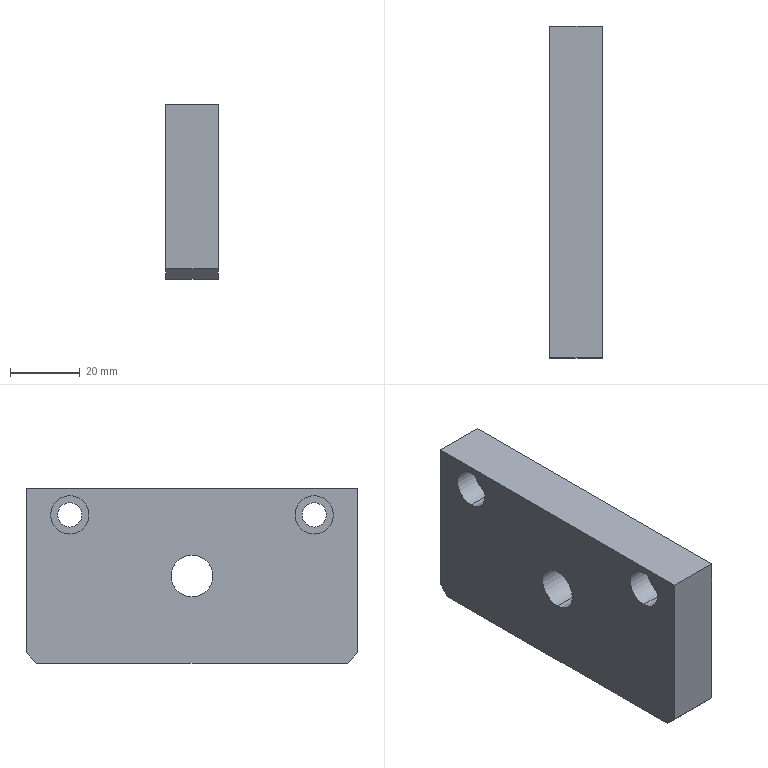Component | SolidWorks | -TighteningHandwheelBasePlate-2 | 1 solid | 20 faces | box 15 x 95 x 50 mm | volume 67472 mm3 | cylinder 10 | plane 10 | commonest cylinder face diameters 11 x4 7 x4 12 x2
build123d program:
from build123d import *

# Parameters (mm, degrees)
SKETCH1_W                                           = 50
SKETCH1_H                                           = 95
BOSS_EXTRUDE1_DEPTH                                 = 15
SKETCH2_R                                           = 6
CUT_EXTRUDE1_DEPTH                                  = 56.734
CYLINDRICAL_COUNTERSUNK_HOLE_FOR_M6_HEX_D           = 7
CYLINDRICAL_COUNTERSUNK_HOLE_FOR_M6_HEX_CBORE_D     = 11
CYLINDRICAL_COUNTERSUNK_HOLE_FOR_M6_HEX_CBORE_DEPTH = 7
CHAMFER1_SIZE                                       = 3


with BuildPart() as part:
    # Sketch1 → Boss-Extrude1 (new body)
    with BuildSketch(Plane.XY):
        Rectangle(SKETCH1_W, SKETCH1_H)
    extrude(amount=BOSS_EXTRUDE1_DEPTH)

    # Sketch2 → Cut-Extrude1 (cut, through all)
    with BuildSketch(Plane.XY.offset(15)):
        Circle(SKETCH2_R)
    extrude(amount=-CUT_EXTRUDE1_DEPTH, mode=Mode.SUBTRACT)

    # Cylindrical Countersunk Hole for M6 Hex (through all)
    with Locations(Plane.XY.offset(15)):
        with Locations((-17.5, 35), (-17.5, -35)):
            CounterBoreHole(CYLINDRICAL_COUNTERSUNK_HOLE_FOR_M6_HEX_D / 2, CYLINDRICAL_COUNTERSUNK_HOLE_FOR_M6_HEX_CBORE_D / 2, CYLINDRICAL_COUNTERSUNK_HOLE_FOR_M6_HEX_CBORE_DEPTH)

    # Chamfer1
    chamfer1_edges = [part.edges().sort_by_distance(p)[0] for p in [
        (25, -47.5, 7.5),
        (25, 47.5, 7.5),
    ]]
    chamfer(chamfer1_edges, length=CHAMFER1_SIZE)


solid = part.part

# Placed as in the assembly
solid = solid.moved(Location((-260, 1239.5, -20), (180, -90, 0)))
STEP:
#1=COLOUR_RGB('',0.7922,0.8196,0.9333);
#2=FILL_AREA_STYLE_COLOUR('',#1);
#3=FILL_AREA_STYLE('',(#2));
#4=SURFACE_STYLE_FILL_AREA(#3);
#5=SURFACE_SIDE_STYLE('',(#4));
#6=SURFACE_STYLE_USAGE(.BOTH.,#5);
#7=PRESENTATION_STYLE_ASSIGNMENT((#6));
#8=CARTESIAN_POINT('',(-10.551,47.421,0.1181));
#9=VERTEX_POINT('',#8);
#10=CARTESIAN_POINT('',(-10.551,47.421,-0.315));
#11=VERTEX_POINT('',#10);
#12=CARTESIAN_POINT('',(-10.551,47.421,-0.09843));
#13=DIRECTION('',(-1.,-0.,0.));
#14=DIRECTION('',(0.,0.,-1.));
#15=AXIS2_PLACEMENT_3D('',#12,#13,#14);
#16=CIRCLE('',#15,0.2165);
#17=EDGE_CURVE('',#9,#11,#16,.T.);
#18=ORIENTED_EDGE('',*,*,#17,.F.);
#19=CARTESIAN_POINT('',(-10.827,47.421,0.1181));
#20=VERTEX_POINT('',#19);
#21=CARTESIAN_POINT('',(-10.827,47.421,0.1181));
#22=DIRECTION('',(-1.,-0.,0.));
#23=VECTOR('',#22,39.37);
#24=LINE('',#21,#23);
#25=EDGE_CURVE('',#9,#20,#24,.T.);
#26=ORIENTED_EDGE('',*,*,#25,.T.);
#27=CARTESIAN_POINT('',(-10.827,47.421,-0.315));
#28=VERTEX_POINT('',#27);
#29=CARTESIAN_POINT('',(-10.827,47.421,-0.09843));
#30=DIRECTION('',(-1.,-0.,0.));
#31=DIRECTION('',(0.,0.,-1.));
#32=AXIS2_PLACEMENT_3D('',#29,#30,#31);
#33=CIRCLE('',#32,0.2165);
#34=EDGE_CURVE('',#20,#28,#33,.T.);
#35=ORIENTED_EDGE('',*,*,#34,.T.);
#36=CARTESIAN_POINT('',(-10.827,47.421,-0.315));
#37=DIRECTION('',(-1.,-0.,0.));
#38=VECTOR('',#37,39.37);
#39=LINE('',#36,#38);
#40=EDGE_CURVE('',#11,#28,#39,.T.);
#41=ORIENTED_EDGE('',*,*,#40,.F.);
#42=EDGE_LOOP('',(#18,#26,#35,#41));
#43=FACE_OUTER_BOUND('',#42,.T.);
#44=CARTESIAN_POINT('',(-10.827,47.421,-0.09843));
#45=DIRECTION('',(-1.,-0.,0.));
#46=DIRECTION('',(0.,0.,-1.));
#47=AXIS2_PLACEMENT_3D('',#44,#45,#46);
#48=CYLINDRICAL_SURFACE('',#47,0.2165);
#49=ADVANCED_FACE('',(#43),#48,.F.);
#50=CARTESIAN_POINT('',(-10.236,47.421,0.03937));
#51=VERTEX_POINT('',#50);
#52=CARTESIAN_POINT('',(-10.236,47.421,-0.2362));
#53=VERTEX_POINT('',#52);
#54=CARTESIAN_POINT('',(-10.236,47.421,-0.09843));
#55=DIRECTION('',(-1.,-0.,0.));
#56=DIRECTION('',(0.,0.,-1.));
#57=AXIS2_PLACEMENT_3D('',#54,#55,#56);
#58=CIRCLE('',#57,0.1378);
#59=EDGE_CURVE('',#51,#53,#58,.T.);
#60=ORIENTED_EDGE('',*,*,#59,.F.);
#61=CARTESIAN_POINT('',(-10.551,47.421,0.03937));
#62=VERTEX_POINT('',#61);
#63=CARTESIAN_POINT('',(-10.827,47.421,0.03937));
#64=DIRECTION('',(-1.,-0.,0.));
#65=VECTOR('',#64,39.37);
#66=LINE('',#63,#65);
#67=EDGE_CURVE('',#51,#62,#66,.T.);
#68=ORIENTED_EDGE('',*,*,#67,.T.);
#69=CARTESIAN_POINT('',(-10.551,47.421,-0.2362));
#70=VERTEX_POINT('',#69);
#71=CARTESIAN_POINT('',(-10.551,47.421,-0.09843));
#72=DIRECTION('',(-1.,-0.,0.));
#73=DIRECTION('',(0.,0.,-1.));
#74=AXIS2_PLACEMENT_3D('',#71,#72,#73);
#75=CIRCLE('',#74,0.1378);
#76=EDGE_CURVE('',#62,#70,#75,.T.);
#77=ORIENTED_EDGE('',*,*,#76,.T.);
#78=CARTESIAN_POINT('',(-10.827,47.421,-0.2362));
#79=DIRECTION('',(-1.,-0.,0.));
#80=VECTOR('',#79,39.37);
#81=LINE('',#78,#80);
#82=EDGE_CURVE('',#53,#70,#81,.T.);
#83=ORIENTED_EDGE('',*,*,#82,.F.);
#84=EDGE_LOOP('',(#60,#68,#77,#83));
#85=FACE_OUTER_BOUND('',#84,.T.);
#86=CARTESIAN_POINT('',(-10.827,47.421,-0.09843));
#87=DIRECTION('',(-1.,-0.,0.));
#88=DIRECTION('',(0.,0.,-1.));
#89=AXIS2_PLACEMENT_3D('',#86,#87,#88);
#90=CYLINDRICAL_SURFACE('',#89,0.1378);
#91=ADVANCED_FACE('',(#85),#90,.F.);
#92=CARTESIAN_POINT('',(-10.551,50.177,0.1181));
#93=VERTEX_POINT('',#92);
#94=CARTESIAN_POINT('',(-10.551,50.177,-0.315));
#95=VERTEX_POINT('',#94);
#96=CARTESIAN_POINT('',(-10.551,50.177,-0.09843));
#97=DIRECTION('',(-1.,-0.,0.));
#98=DIRECTION('',(0.,0.,-1.));
#99=AXIS2_PLACEMENT_3D('',#96,#97,#98);
#100=CIRCLE('',#99,0.2165);
#101=EDGE_CURVE('',#93,#95,#100,.T.);
#102=ORIENTED_EDGE('',*,*,#101,.F.);
#103=CARTESIAN_POINT('',(-10.827,50.177,0.1181));
#104=VERTEX_POINT('',#103);
#105=CARTESIAN_POINT('',(-10.827,50.177,0.1181));
#106=DIRECTION('',(-1.,-0.,0.));
#107=VECTOR('',#106,39.37);
#108=LINE('',#105,#107);
#109=EDGE_CURVE('',#93,#104,#108,.T.);
#110=ORIENTED_EDGE('',*,*,#109,.T.);
#111=CARTESIAN_POINT('',(-10.827,50.177,-0.315));
#112=VERTEX_POINT('',#111);
#113=CARTESIAN_POINT('',(-10.827,50.177,-0.09843));
#114=DIRECTION('',(-1.,-0.,0.));
#115=DIRECTION('',(0.,0.,-1.));
#116=AXIS2_PLACEMENT_3D('',#113,#114,#115);
#117=CIRCLE('',#116,0.2165);
#118=EDGE_CURVE('',#104,#112,#117,.T.);
#119=ORIENTED_EDGE('',*,*,#118,.T.);
#120=CARTESIAN_POINT('',(-10.827,50.177,-0.315));
#121=DIRECTION('',(-1.,-0.,0.));
#122=VECTOR('',#121,39.37);
#123=LINE('',#120,#122);
#124=EDGE_CURVE('',#95,#112,#123,.T.);
#125=ORIENTED_EDGE('',*,*,#124,.F.);
#126=EDGE_LOOP('',(#102,#110,#119,#125));
#127=FACE_OUTER_BOUND('',#126,.T.);
#128=CARTESIAN_POINT('',(-10.827,50.177,-0.09843));
#129=DIRECTION('',(-1.,-0.,0.));
#130=DIRECTION('',(0.,0.,-1.));
#131=AXIS2_PLACEMENT_3D('',#128,#129,#130);
#132=CYLINDRICAL_SURFACE('',#131,0.2165);
#133=ADVANCED_FACE('',(#127),#132,.F.);
#134=CARTESIAN_POINT('',(-10.236,50.177,0.03937));
#135=VERTEX_POINT('',#134);
#136=CARTESIAN_POINT('',(-10.236,50.177,-0.2362));
#137=VERTEX_POINT('',#136);
#138=CARTESIAN_POINT('',(-10.236,50.177,-0.09843));
#139=DIRECTION('',(-1.,-0.,0.));
#140=DIRECTION('',(0.,0.,-1.));
#141=AXIS2_PLACEMENT_3D('',#138,#139,#140);
#142=CIRCLE('',#141,0.1378);
#143=EDGE_CURVE('',#135,#137,#142,.T.);
#144=ORIENTED_EDGE('',*,*,#143,.F.);
#145=CARTESIAN_POINT('',(-10.551,50.177,0.03937));
#146=VERTEX_POINT('',#145);
#147=CARTESIAN_POINT('',(-10.827,50.177,0.03937));
#148=DIRECTION('',(-1.,-0.,0.));
#149=VECTOR('',#148,39.37);
#150=LINE('',#147,#149);
#151=EDGE_CURVE('',#135,#146,#150,.T.);
#152=ORIENTED_EDGE('',*,*,#151,.T.);
#153=CARTESIAN_POINT('',(-10.551,50.177,-0.2362));
#154=VERTEX_POINT('',#153);
#155=CARTESIAN_POINT('',(-10.551,50.177,-0.09843));
#156=DIRECTION('',(-1.,-0.,0.));
#157=DIRECTION('',(0.,0.,-1.));
#158=AXIS2_PLACEMENT_3D('',#155,#156,#157);
#159=CIRCLE('',#158,0.1378);
#160=EDGE_CURVE('',#146,#154,#159,.T.);
#161=ORIENTED_EDGE('',*,*,#160,.T.);
#162=CARTESIAN_POINT('',(-10.827,50.177,-0.2362));
#163=DIRECTION('',(-1.,-0.,0.));
#164=VECTOR('',#163,39.37);
#165=LINE('',#162,#164);
#166=EDGE_CURVE('',#137,#154,#165,.T.);
#167=ORIENTED_EDGE('',*,*,#166,.F.);
#168=EDGE_LOOP('',(#144,#152,#161,#167));
#169=FACE_OUTER_BOUND('',#168,.T.);
#170=CARTESIAN_POINT('',(-10.827,50.177,-0.09843));
#171=DIRECTION('',(-1.,-0.,0.));
#172=DIRECTION('',(0.,0.,-1.));
#173=AXIS2_PLACEMENT_3D('',#170,#171,#172);
#174=CYLINDRICAL_SURFACE('',#173,0.1378);
#175=ADVANCED_FACE('',(#169),#174,.F.);
#176=CARTESIAN_POINT('',(-10.236,48.799,-0.5512));
#177=VERTEX_POINT('',#176);
#178=CARTESIAN_POINT('',(-10.236,48.799,-1.024));
#179=VERTEX_POINT('',#178);
#180=CARTESIAN_POINT('',(-10.236,48.799,-0.7874));
#181=DIRECTION('',(-1.,-0.,0.));
#182=DIRECTION('',(0.,0.,-1.));
#183=AXIS2_PLACEMENT_3D('',#180,#181,#182);
#184=CIRCLE('',#183,0.2362);
#185=EDGE_CURVE('',#177,#179,#184,.T.);
#186=ORIENTED_EDGE('',*,*,#185,.F.);
#187=CARTESIAN_POINT('',(-10.827,48.799,-0.5512));
#188=VERTEX_POINT('',#187);
#189=CARTESIAN_POINT('',(-10.236,48.799,-0.5512));
#190=DIRECTION('',(-1.,-0.,0.));
#191=VECTOR('',#190,39.37);
#192=LINE('',#189,#191);
#193=EDGE_CURVE('',#177,#188,#192,.T.);
#194=ORIENTED_EDGE('',*,*,#193,.T.);
#195=CARTESIAN_POINT('',(-10.827,48.799,-1.024));
#196=VERTEX_POINT('',#195);
#197=CARTESIAN_POINT('',(-10.827,48.799,-0.7874));
#198=DIRECTION('',(-1.,-0.,0.));
#199=DIRECTION('',(0.,0.,-1.));
#200=AXIS2_PLACEMENT_3D('',#197,#198,#199);
#201=CIRCLE('',#200,0.2362);
#202=EDGE_CURVE('',#188,#196,#201,.T.);
#203=ORIENTED_EDGE('',*,*,#202,.T.);
#204=CARTESIAN_POINT('',(-10.236,48.799,-1.024));
#205=DIRECTION('',(-1.,-0.,0.));
#206=VECTOR('',#205,39.37);
#207=LINE('',#204,#206);
#208=EDGE_CURVE('',#179,#196,#207,.T.);
#209=ORIENTED_EDGE('',*,*,#208,.F.);
#210=EDGE_LOOP('',(#186,#194,#203,#209));
#211=FACE_OUTER_BOUND('',#210,.T.);
#212=CARTESIAN_POINT('',(-10.236,48.799,-0.7874));
#213=DIRECTION('',(-1.,-0.,0.));
#214=DIRECTION('',(0.,0.,-1.));
#215=AXIS2_PLACEMENT_3D('',#212,#213,#214);
#216=CYLINDRICAL_SURFACE('',#215,0.2362);
#217=ADVANCED_FACE('',(#211),#216,.F.);
#218=CARTESIAN_POINT('',(-10.827,50.551,-1.772));
#219=VERTEX_POINT('',#218);
#220=CARTESIAN_POINT('',(-10.827,47.047,-1.772));
#221=VERTEX_POINT('',#220);
#222=CARTESIAN_POINT('',(-10.827,46.929,-1.772));
#223=DIRECTION('',(0.,-1.,0.));
#224=VECTOR('',#223,39.37);
#225=LINE('',#222,#224);
#226=EDGE_CURVE('',#219,#221,#225,.T.);
#227=ORIENTED_EDGE('',*,*,#226,.F.);
#228=CARTESIAN_POINT('',(-10.236,50.551,-1.772));
#229=VERTEX_POINT('',#228);
#230=CARTESIAN_POINT('',(-10.827,50.551,-1.772));
#231=DIRECTION('',(1.,0.,-0.));
#232=VECTOR('',#231,39.37);
#233=LINE('',#230,#232);
#234=EDGE_CURVE('',#219,#229,#233,.T.);
#235=ORIENTED_EDGE('',*,*,#234,.T.);
#236=CARTESIAN_POINT('',(-10.236,47.047,-1.772));
#237=VERTEX_POINT('',#236);
#238=CARTESIAN_POINT('',(-10.236,46.929,-1.772));
#239=DIRECTION('',(0.,-1.,0.));
#240=VECTOR('',#239,39.37);
#241=LINE('',#238,#240);
#242=EDGE_CURVE('',#229,#237,#241,.T.);
#243=ORIENTED_EDGE('',*,*,#242,.T.);
#244=CARTESIAN_POINT('',(-10.827,47.047,-1.772));
#245=DIRECTION('',(-1.,-0.,0.));
#246=VECTOR('',#245,39.37);
#247=LINE('',#244,#246);
#248=EDGE_CURVE('',#237,#221,#247,.T.);
#249=ORIENTED_EDGE('',*,*,#248,.T.);
#250=EDGE_LOOP('',(#227,#235,#243,#249));
#251=FACE_OUTER_BOUND('',#250,.T.);
#252=CARTESIAN_POINT('',(-10.827,46.929,-1.772));
#253=DIRECTION('',(0.,0.,1.));
#254=DIRECTION('',(-0.,1.,-0.));
#255=AXIS2_PLACEMENT_3D('',#252,#253,#254);
#256=PLANE('',#255);
#257=ADVANCED_FACE('',(#251),#256,.F.);
#258=CARTESIAN_POINT('',(-10.827,46.929,-1.654));
#259=VERTEX_POINT('',#258);
#260=CARTESIAN_POINT('',(-10.827,46.929,0.1969));
#261=VERTEX_POINT('',#260);
#262=CARTESIAN_POINT('',(-10.827,46.929,0.1969));
#263=DIRECTION('',(0.,-0.,1.));
#264=VECTOR('',#263,39.37);
#265=LINE('',#262,#264);
#266=EDGE_CURVE('',#259,#261,#265,.T.);
#267=ORIENTED_EDGE('',*,*,#266,.F.);
#268=CARTESIAN_POINT('',(-10.236,46.929,-1.654));
#269=VERTEX_POINT('',#268);
#270=CARTESIAN_POINT('',(-10.827,46.929,-1.654));
#271=DIRECTION('',(1.,0.,-0.));
#272=VECTOR('',#271,39.37);
#273=LINE('',#270,#272);
#274=EDGE_CURVE('',#259,#269,#273,.T.);
#275=ORIENTED_EDGE('',*,*,#274,.T.);
#276=CARTESIAN_POINT('',(-10.236,46.929,0.1969));
#277=VERTEX_POINT('',#276);
#278=CARTESIAN_POINT('',(-10.236,46.929,0.1969));
#279=DIRECTION('',(0.,-0.,1.));
#280=VECTOR('',#279,39.37);
#281=LINE('',#278,#280);
#282=EDGE_CURVE('',#269,#277,#281,.T.);
#283=ORIENTED_EDGE('',*,*,#282,.T.);
#284=CARTESIAN_POINT('',(-10.827,46.929,0.1969));
#285=DIRECTION('',(1.,0.,-0.));
#286=VECTOR('',#285,39.37);
#287=LINE('',#284,#286);
#288=EDGE_CURVE('',#261,#277,#287,.T.);
#289=ORIENTED_EDGE('',*,*,#288,.F.);
#290=EDGE_LOOP('',(#267,#275,#283,#289));
#291=FACE_OUTER_BOUND('',#290,.T.);
#292=CARTESIAN_POINT('',(-10.827,46.929,0.1969));
#293=DIRECTION('',(-0.,1.,0.));
#294=DIRECTION('',(1.,0.,-0.));
#295=AXIS2_PLACEMENT_3D('',#292,#293,#294);
#296=PLANE('',#295);
#297=ADVANCED_FACE('',(#291),#296,.F.);
#298=CARTESIAN_POINT('',(-10.236,50.669,0.1969));
#299=VERTEX_POINT('',#298);
#300=CARTESIAN_POINT('',(-10.236,46.929,0.1969));
#301=DIRECTION('',(-0.,1.,-0.));
#302=VECTOR('',#301,39.37);
#303=LINE('',#300,#302);
#304=EDGE_CURVE('',#277,#299,#303,.T.);
#305=ORIENTED_EDGE('',*,*,#304,.T.);
#306=CARTESIAN_POINT('',(-10.827,50.669,0.1969));
#307=VERTEX_POINT('',#306);
#308=CARTESIAN_POINT('',(-10.827,50.669,0.1969));
#309=DIRECTION('',(1.,0.,-0.));
#310=VECTOR('',#309,39.37);
#311=LINE('',#308,#310);
#312=EDGE_CURVE('',#307,#299,#311,.T.);
#313=ORIENTED_EDGE('',*,*,#312,.F.);
#314=CARTESIAN_POINT('',(-10.827,46.929,0.1969));
#315=DIRECTION('',(-0.,1.,-0.));
#316=VECTOR('',#315,39.37);
#317=LINE('',#314,#316);
#318=EDGE_CURVE('',#261,#307,#317,.T.);
#319=ORIENTED_EDGE('',*,*,#318,.F.);
#320=ORIENTED_EDGE('',*,*,#288,.T.);
#321=EDGE_LOOP('',(#305,#313,#319,#320));
#322=FACE_OUTER_BOUND('',#321,.T.);
#323=CARTESIAN_POINT('',(-10.827,46.929,0.1969));
#324=DIRECTION('',(-0.,-0.,-1.));
#325=DIRECTION('',(0.,-1.,0.));
#326=AXIS2_PLACEMENT_3D('',#323,#324,#325);
#327=PLANE('',#326);
#328=ADVANCED_FACE('',(#322),#327,.F.);
#329=CARTESIAN_POINT('',(-10.236,50.669,-1.654));
#330=VERTEX_POINT('',#329);
#331=CARTESIAN_POINT('',(-10.236,50.669,0.1969));
#332=DIRECTION('',(-0.,0.,-1.));
#333=VECTOR('',#332,39.37);
#334=LINE('',#331,#333);
#335=EDGE_CURVE('',#299,#330,#334,.T.);
#336=ORIENTED_EDGE('',*,*,#335,.T.);
#337=CARTESIAN_POINT('',(-10.827,50.669,-1.654));
#338=VERTEX_POINT('',#337);
#339=CARTESIAN_POINT('',(-10.827,50.669,-1.654));
#340=DIRECTION('',(-1.,-0.,0.));
#341=VECTOR('',#340,39.37);
#342=LINE('',#339,#341);
#343=EDGE_CURVE('',#330,#338,#342,.T.);
#344=ORIENTED_EDGE('',*,*,#343,.T.);
#345=CARTESIAN_POINT('',(-10.827,50.669,0.1969));
#346=DIRECTION('',(-0.,0.,-1.));
#347=VECTOR('',#346,39.37);
#348=LINE('',#345,#347);
#349=EDGE_CURVE('',#307,#338,#348,.T.);
#350=ORIENTED_EDGE('',*,*,#349,.F.);
#351=ORIENTED_EDGE('',*,*,#312,.T.);
#352=EDGE_LOOP('',(#336,#344,#350,#351));
#353=FACE_OUTER_BOUND('',#352,.T.);
#354=CARTESIAN_POINT('',(-10.827,50.669,0.1969));
#355=DIRECTION('',(0.,-1.,-0.));
#356=DIRECTION('',(-1.,-0.,0.));
#357=AXIS2_PLACEMENT_3D('',#354,#355,#356);
#358=PLANE('',#357);
#359=ADVANCED_FACE('',(#353),#358,.F.);
#360=CARTESIAN_POINT('',(-10.827,47.421,-0.09843));
#361=DIRECTION('',(-1.,-0.,0.));
#362=DIRECTION('',(0.,0.,-1.));
#363=AXIS2_PLACEMENT_3D('',#360,#361,#362);
#364=CIRCLE('',#363,0.2165);
#365=EDGE_CURVE('',#28,#20,#364,.T.);
#366=ORIENTED_EDGE('',*,*,#365,.F.);
#367=ORIENTED_EDGE('',*,*,#34,.F.);
#368=EDGE_LOOP('',(#366,#367));
#369=FACE_BOUND('',#368,.T.);
#370=CARTESIAN_POINT('',(-10.827,50.177,-0.09843));
#371=DIRECTION('',(-1.,-0.,0.));
#372=DIRECTION('',(0.,0.,-1.));
#373=AXIS2_PLACEMENT_3D('',#370,#371,#372);
#374=CIRCLE('',#373,0.2165);
#375=EDGE_CURVE('',#112,#104,#374,.T.);
#376=ORIENTED_EDGE('',*,*,#375,.F.);
#377=ORIENTED_EDGE('',*,*,#118,.F.);
#378=EDGE_LOOP('',(#376,#377));
#379=FACE_BOUND('',#378,.T.);
#380=CARTESIAN_POINT('',(-10.827,48.799,-0.7874));
#381=DIRECTION('',(-1.,-0.,0.));
#382=DIRECTION('',(0.,0.,-1.));
#383=AXIS2_PLACEMENT_3D('',#380,#381,#382);
#384=CIRCLE('',#383,0.2362);
#385=EDGE_CURVE('',#196,#188,#384,.T.);
#386=ORIENTED_EDGE('',*,*,#385,.F.);
#387=ORIENTED_EDGE('',*,*,#202,.F.);
#388=EDGE_LOOP('',(#386,#387));
#389=FACE_BOUND('',#388,.T.);
#390=ORIENTED_EDGE('',*,*,#349,.T.);
#391=CARTESIAN_POINT('',(-10.827,50.167,-2.156));
#392=DIRECTION('',(0.,-0.7071,-0.7071));
#393=VECTOR('',#392,39.37);
#394=LINE('',#391,#393);
#395=EDGE_CURVE('',#338,#219,#394,.T.);
#396=ORIENTED_EDGE('',*,*,#395,.T.);
#397=ORIENTED_EDGE('',*,*,#226,.T.);
#398=CARTESIAN_POINT('',(-10.827,47.431,-2.156));
#399=DIRECTION('',(0.,-0.7071,0.7071));
#400=VECTOR('',#399,39.37);
#401=LINE('',#398,#400);
#402=EDGE_CURVE('',#221,#259,#401,.T.);
#403=ORIENTED_EDGE('',*,*,#402,.T.);
#404=ORIENTED_EDGE('',*,*,#266,.T.);
#405=ORIENTED_EDGE('',*,*,#318,.T.);
#406=EDGE_LOOP('',(#390,#396,#397,#403,#404,#405));
#407=FACE_OUTER_BOUND('',#406,.T.);
#408=CARTESIAN_POINT('',(-10.827,48.799,-0.7874));
#409=DIRECTION('',(-1.,-0.,0.));
#410=DIRECTION('',(-0.,0.,-1.));
#411=AXIS2_PLACEMENT_3D('',#408,#409,#410);
#412=PLANE('',#411);
#413=ADVANCED_FACE('',(#369,#379,#389,#407),#412,.T.);
#414=CARTESIAN_POINT('',(-10.236,47.421,-0.09843));
#415=DIRECTION('',(-1.,-0.,0.));
#416=DIRECTION('',(0.,0.,-1.));
#417=AXIS2_PLACEMENT_3D('',#414,#415,#416);
#418=CIRCLE('',#417,0.1378);
#419=EDGE_CURVE('',#53,#51,#418,.T.);
#420=ORIENTED_EDGE('',*,*,#419,.T.);
#421=ORIENTED_EDGE('',*,*,#59,.T.);
#422=EDGE_LOOP('',(#420,#421));
#423=FACE_BOUND('',#422,.T.);
#424=CARTESIAN_POINT('',(-10.236,50.177,-0.09843));
#425=DIRECTION('',(-1.,-0.,0.));
#426=DIRECTION('',(0.,0.,-1.));
#427=AXIS2_PLACEMENT_3D('',#424,#425,#426);
#428=CIRCLE('',#427,0.1378);
#429=EDGE_CURVE('',#137,#135,#428,.T.);
#430=ORIENTED_EDGE('',*,*,#429,.T.);
#431=ORIENTED_EDGE('',*,*,#143,.T.);
#432=EDGE_LOOP('',(#430,#431));
#433=FACE_BOUND('',#432,.T.);
#434=CARTESIAN_POINT('',(-10.236,48.799,-0.7874));
#435=DIRECTION('',(-1.,-0.,0.));
#436=DIRECTION('',(0.,0.,-1.));
#437=AXIS2_PLACEMENT_3D('',#434,#435,#436);
#438=CIRCLE('',#437,0.2362);
#439=EDGE_CURVE('',#179,#177,#438,.T.);
#440=ORIENTED_EDGE('',*,*,#439,.T.);
#441=ORIENTED_EDGE('',*,*,#185,.T.);
#442=EDGE_LOOP('',(#440,#441));
#443=FACE_BOUND('',#442,.T.);
#444=ORIENTED_EDGE('',*,*,#242,.F.);
#445=CARTESIAN_POINT('',(-10.236,50.551,-1.772));
#446=DIRECTION('',(-0.,0.7071,0.7071));
#447=VECTOR('',#446,39.37);
#448=LINE('',#445,#447);
#449=EDGE_CURVE('',#229,#330,#448,.T.);
#450=ORIENTED_EDGE('',*,*,#449,.T.);
#451=ORIENTED_EDGE('',*,*,#335,.F.);
#452=ORIENTED_EDGE('',*,*,#304,.F.);
#453=ORIENTED_EDGE('',*,*,#282,.F.);
#454=CARTESIAN_POINT('',(-10.236,46.929,-1.654));
#455=DIRECTION('',(-0.,0.7071,-0.7071));
#456=VECTOR('',#455,39.37);
#457=LINE('',#454,#456);
#458=EDGE_CURVE('',#269,#237,#457,.T.);
#459=ORIENTED_EDGE('',*,*,#458,.T.);
#460=EDGE_LOOP('',(#444,#450,#451,#452,#453,#459));
#461=FACE_OUTER_BOUND('',#460,.T.);
#462=CARTESIAN_POINT('',(-10.236,48.799,-0.7874));
#463=DIRECTION('',(-1.,-0.,0.));
#464=DIRECTION('',(-0.,0.,-1.));
#465=AXIS2_PLACEMENT_3D('',#462,#463,#464);
#466=PLANE('',#465);
#467=ADVANCED_FACE('',(#423,#433,#443,#461),#466,.F.);
#468=ORIENTED_EDGE('',*,*,#193,.F.);
#469=ORIENTED_EDGE('',*,*,#439,.F.);
#470=ORIENTED_EDGE('',*,*,#208,.T.);
#471=ORIENTED_EDGE('',*,*,#385,.T.);
#472=EDGE_LOOP('',(#468,#469,#470,#471));
#473=FACE_OUTER_BOUND('',#472,.T.);
#474=CARTESIAN_POINT('',(-10.236,48.799,-0.7874));
#475=DIRECTION('',(-1.,-0.,0.));
#476=DIRECTION('',(0.,0.,-1.));
#477=AXIS2_PLACEMENT_3D('',#474,#475,#476);
#478=CYLINDRICAL_SURFACE('',#477,0.2362);
#479=ADVANCED_FACE('',(#473),#478,.F.);
#480=ORIENTED_EDGE('',*,*,#151,.F.);
#481=ORIENTED_EDGE('',*,*,#429,.F.);
#482=ORIENTED_EDGE('',*,*,#166,.T.);
#483=CARTESIAN_POINT('',(-10.551,50.177,-0.09843));
#484=DIRECTION('',(-1.,-0.,0.));
#485=DIRECTION('',(0.,0.,-1.));
#486=AXIS2_PLACEMENT_3D('',#483,#484,#485);
#487=CIRCLE('',#486,0.1378);
#488=EDGE_CURVE('',#154,#146,#487,.T.);
#489=ORIENTED_EDGE('',*,*,#488,.T.);
#490=EDGE_LOOP('',(#480,#481,#482,#489));
#491=FACE_OUTER_BOUND('',#490,.T.);
#492=CARTESIAN_POINT('',(-10.827,50.177,-0.09843));
#493=DIRECTION('',(-1.,-0.,0.));
#494=DIRECTION('',(0.,0.,-1.));
#495=AXIS2_PLACEMENT_3D('',#492,#493,#494);
#496=CYLINDRICAL_SURFACE('',#495,0.1378);
#497=ADVANCED_FACE('',(#491),#496,.F.);
#498=ORIENTED_EDGE('',*,*,#488,.F.);
#499=ORIENTED_EDGE('',*,*,#160,.F.);
#500=EDGE_LOOP('',(#498,#499));
#501=FACE_BOUND('',#500,.T.);
#502=CARTESIAN_POINT('',(-10.551,50.177,-0.09843));
#503=DIRECTION('',(-1.,-0.,0.));
#504=DIRECTION('',(0.,0.,-1.));
#505=AXIS2_PLACEMENT_3D('',#502,#503,#504);
#506=CIRCLE('',#505,0.2165);
#507=EDGE_CURVE('',#95,#93,#506,.T.);
#508=ORIENTED_EDGE('',*,*,#507,.T.);
#509=ORIENTED_EDGE('',*,*,#101,.T.);
#510=EDGE_LOOP('',(#508,#509));
#511=FACE_OUTER_BOUND('',#510,.T.);
#512=CARTESIAN_POINT('',(-10.551,50.177,-0.2362));
#513=DIRECTION('',(1.,0.,-0.));
#514=DIRECTION('',(0.,-0.,1.));
#515=AXIS2_PLACEMENT_3D('',#512,#513,#514);
#516=PLANE('',#515);
#517=ADVANCED_FACE('',(#501,#511),#516,.F.);
#518=ORIENTED_EDGE('',*,*,#109,.F.);
#519=ORIENTED_EDGE('',*,*,#507,.F.);
#520=ORIENTED_EDGE('',*,*,#124,.T.);
#521=ORIENTED_EDGE('',*,*,#375,.T.);
#522=EDGE_LOOP('',(#518,#519,#520,#521));
#523=FACE_OUTER_BOUND('',#522,.T.);
#524=CARTESIAN_POINT('',(-10.827,50.177,-0.09843));
#525=DIRECTION('',(-1.,-0.,0.));
#526=DIRECTION('',(0.,0.,-1.));
#527=AXIS2_PLACEMENT_3D('',#524,#525,#526);
#528=CYLINDRICAL_SURFACE('',#527,0.2165);
#529=ADVANCED_FACE('',(#523),#528,.F.);
#530=ORIENTED_EDGE('',*,*,#67,.F.);
#531=ORIENTED_EDGE('',*,*,#419,.F.);
#532=ORIENTED_EDGE('',*,*,#82,.T.);
#533=CARTESIAN_POINT('',(-10.551,47.421,-0.09843));
#534=DIRECTION('',(-1.,-0.,0.));
#535=DIRECTION('',(0.,0.,-1.));
#536=AXIS2_PLACEMENT_3D('',#533,#534,#535);
#537=CIRCLE('',#536,0.1378);
#538=EDGE_CURVE('',#70,#62,#537,.T.);
#539=ORIENTED_EDGE('',*,*,#538,.T.);
#540=EDGE_LOOP('',(#530,#531,#532,#539));
#541=FACE_OUTER_BOUND('',#540,.T.);
#542=CARTESIAN_POINT('',(-10.827,47.421,-0.09843));
#543=DIRECTION('',(-1.,-0.,0.));
#544=DIRECTION('',(0.,0.,-1.));
#545=AXIS2_PLACEMENT_3D('',#542,#543,#544);
#546=CYLINDRICAL_SURFACE('',#545,0.1378);
#547=ADVANCED_FACE('',(#541),#546,.F.);
#548=ORIENTED_EDGE('',*,*,#538,.F.);
#549=ORIENTED_EDGE('',*,*,#76,.F.);
#550=EDGE_LOOP('',(#548,#549));
#551=FACE_BOUND('',#550,.T.);
#552=CARTESIAN_POINT('',(-10.551,47.421,-0.09843));
#553=DIRECTION('',(-1.,-0.,0.));
#554=DIRECTION('',(0.,0.,-1.));
#555=AXIS2_PLACEMENT_3D('',#552,#553,#554);
#556=CIRCLE('',#555,0.2165);
#557=EDGE_CURVE('',#11,#9,#556,.T.);
#558=ORIENTED_EDGE('',*,*,#557,.T.);
#559=ORIENTED_EDGE('',*,*,#17,.T.);
#560=EDGE_LOOP('',(#558,#559));
#561=FACE_OUTER_BOUND('',#560,.T.);
#562=CARTESIAN_POINT('',(-10.551,47.421,-0.2362));
#563=DIRECTION('',(1.,0.,-0.));
#564=DIRECTION('',(0.,-0.,1.));
#565=AXIS2_PLACEMENT_3D('',#562,#563,#564);
#566=PLANE('',#565);
#567=ADVANCED_FACE('',(#551,#561),#566,.F.);
#568=ORIENTED_EDGE('',*,*,#25,.F.);
#569=ORIENTED_EDGE('',*,*,#557,.F.);
#570=ORIENTED_EDGE('',*,*,#40,.T.);
#571=ORIENTED_EDGE('',*,*,#365,.T.);
#572=EDGE_LOOP('',(#568,#569,#570,#571));
#573=FACE_OUTER_BOUND('',#572,.T.);
#574=CARTESIAN_POINT('',(-10.827,47.421,-0.09843));
#575=DIRECTION('',(-1.,-0.,0.));
#576=DIRECTION('',(0.,0.,-1.));
#577=AXIS2_PLACEMENT_3D('',#574,#575,#576);
#578=CYLINDRICAL_SURFACE('',#577,0.2165);
#579=ADVANCED_FACE('',(#573),#578,.F.);
#580=ORIENTED_EDGE('',*,*,#395,.F.);
#581=ORIENTED_EDGE('',*,*,#343,.F.);
#582=ORIENTED_EDGE('',*,*,#449,.F.);
#583=ORIENTED_EDGE('',*,*,#234,.F.);
#584=EDGE_LOOP('',(#580,#581,#582,#583));
#585=FACE_OUTER_BOUND('',#584,.T.);
#586=CARTESIAN_POINT('',(-10.827,50.551,-1.772));
#587=DIRECTION('',(0.,-0.7071,0.7071));
#588=DIRECTION('',(1.,0.,-0.));
#589=AXIS2_PLACEMENT_3D('',#586,#587,#588);
#590=PLANE('',#589);
#591=ADVANCED_FACE('',(#585),#590,.F.);
#592=ORIENTED_EDGE('',*,*,#402,.F.);
#593=ORIENTED_EDGE('',*,*,#248,.F.);
#594=ORIENTED_EDGE('',*,*,#458,.F.);
#595=ORIENTED_EDGE('',*,*,#274,.F.);
#596=EDGE_LOOP('',(#592,#593,#594,#595));
#597=FACE_OUTER_BOUND('',#596,.T.);
#598=CARTESIAN_POINT('',(-10.827,46.929,-1.654));
#599=DIRECTION('',(-0.,0.7071,0.7071));
#600=DIRECTION('',(1.,0.,-0.));
#601=AXIS2_PLACEMENT_3D('',#598,#599,#600);
#602=PLANE('',#601);
#603=ADVANCED_FACE('',(#597),#602,.F.);
#604=CLOSED_SHELL('',(#49,#91,#133,#175,#217,#257,#297,#328,#359,#413,#467,#479,#497,#517,#529,#547,#567,#579,#591,#603));
#605=MANIFOLD_SOLID_BREP('',#604);
#606=STYLED_ITEM('',(#7),#605);
#607=PRESENTATION_LAYER_ASSIGNMENT('','',(#606));
#608=CARTESIAN_POINT('',(0.,0.,0.));
#609=DIRECTION('',(0.,0.,1.));
#610=DIRECTION('',(1.,0.,0.));
#611=AXIS2_PLACEMENT_3D('',#608,#609,#610);
#612=(LENGTH_UNIT()NAMED_UNIT(*)SI_UNIT($,.METRE.));
#613=LENGTH_MEASURE_WITH_UNIT(LENGTH_MEASURE(0.0254),#612);
#614=DIMENSIONAL_EXPONENTS(1.,0.,0.,0.,0.,0.,0.);
#615=(CONVERSION_BASED_UNIT('',#613)LENGTH_UNIT()NAMED_UNIT(#614));
#616=UNCERTAINTY_MEASURE_WITH_UNIT(LENGTH_MEASURE(0.00001),#615,'','');
#617=(NAMED_UNIT(*)PLANE_ANGLE_UNIT()SI_UNIT($,.RADIAN.));
#618=(NAMED_UNIT(*)SI_UNIT($,.STERADIAN.)SOLID_ANGLE_UNIT());
#619=(GEOMETRIC_REPRESENTATION_CONTEXT(3)GLOBAL_UNCERTAINTY_ASSIGNED_CONTEXT((#616))GLOBAL_UNIT_ASSIGNED_CONTEXT((#615,#617,#618))REPRESENTATION_CONTEXT('',''));
#620=ADVANCED_BREP_SHAPE_REPRESENTATION('',(#605,#611),#619);
#621=(LENGTH_UNIT()NAMED_UNIT(*)SI_UNIT($,.METRE.));
#622=LENGTH_MEASURE_WITH_UNIT(LENGTH_MEASURE(0.0254),#621);
#623=DIMENSIONAL_EXPONENTS(1.,0.,0.,0.,0.,0.,0.);
#624=(CONVERSION_BASED_UNIT('',#622)LENGTH_UNIT()NAMED_UNIT(#623));
#625=UNCERTAINTY_MEASURE_WITH_UNIT(LENGTH_MEASURE(0.00001),#624,'','');
#626=(NAMED_UNIT(*)PLANE_ANGLE_UNIT()SI_UNIT($,.RADIAN.));
#627=(NAMED_UNIT(*)SI_UNIT($,.STERADIAN.)SOLID_ANGLE_UNIT());
#628=(GEOMETRIC_REPRESENTATION_CONTEXT(3)GLOBAL_UNCERTAINTY_ASSIGNED_CONTEXT((#625))GLOBAL_UNIT_ASSIGNED_CONTEXT((#624,#626,#627))REPRESENTATION_CONTEXT('',''));
#629=MECHANICAL_DESIGN_GEOMETRIC_PRESENTATION_REPRESENTATION('',(#606),#628);